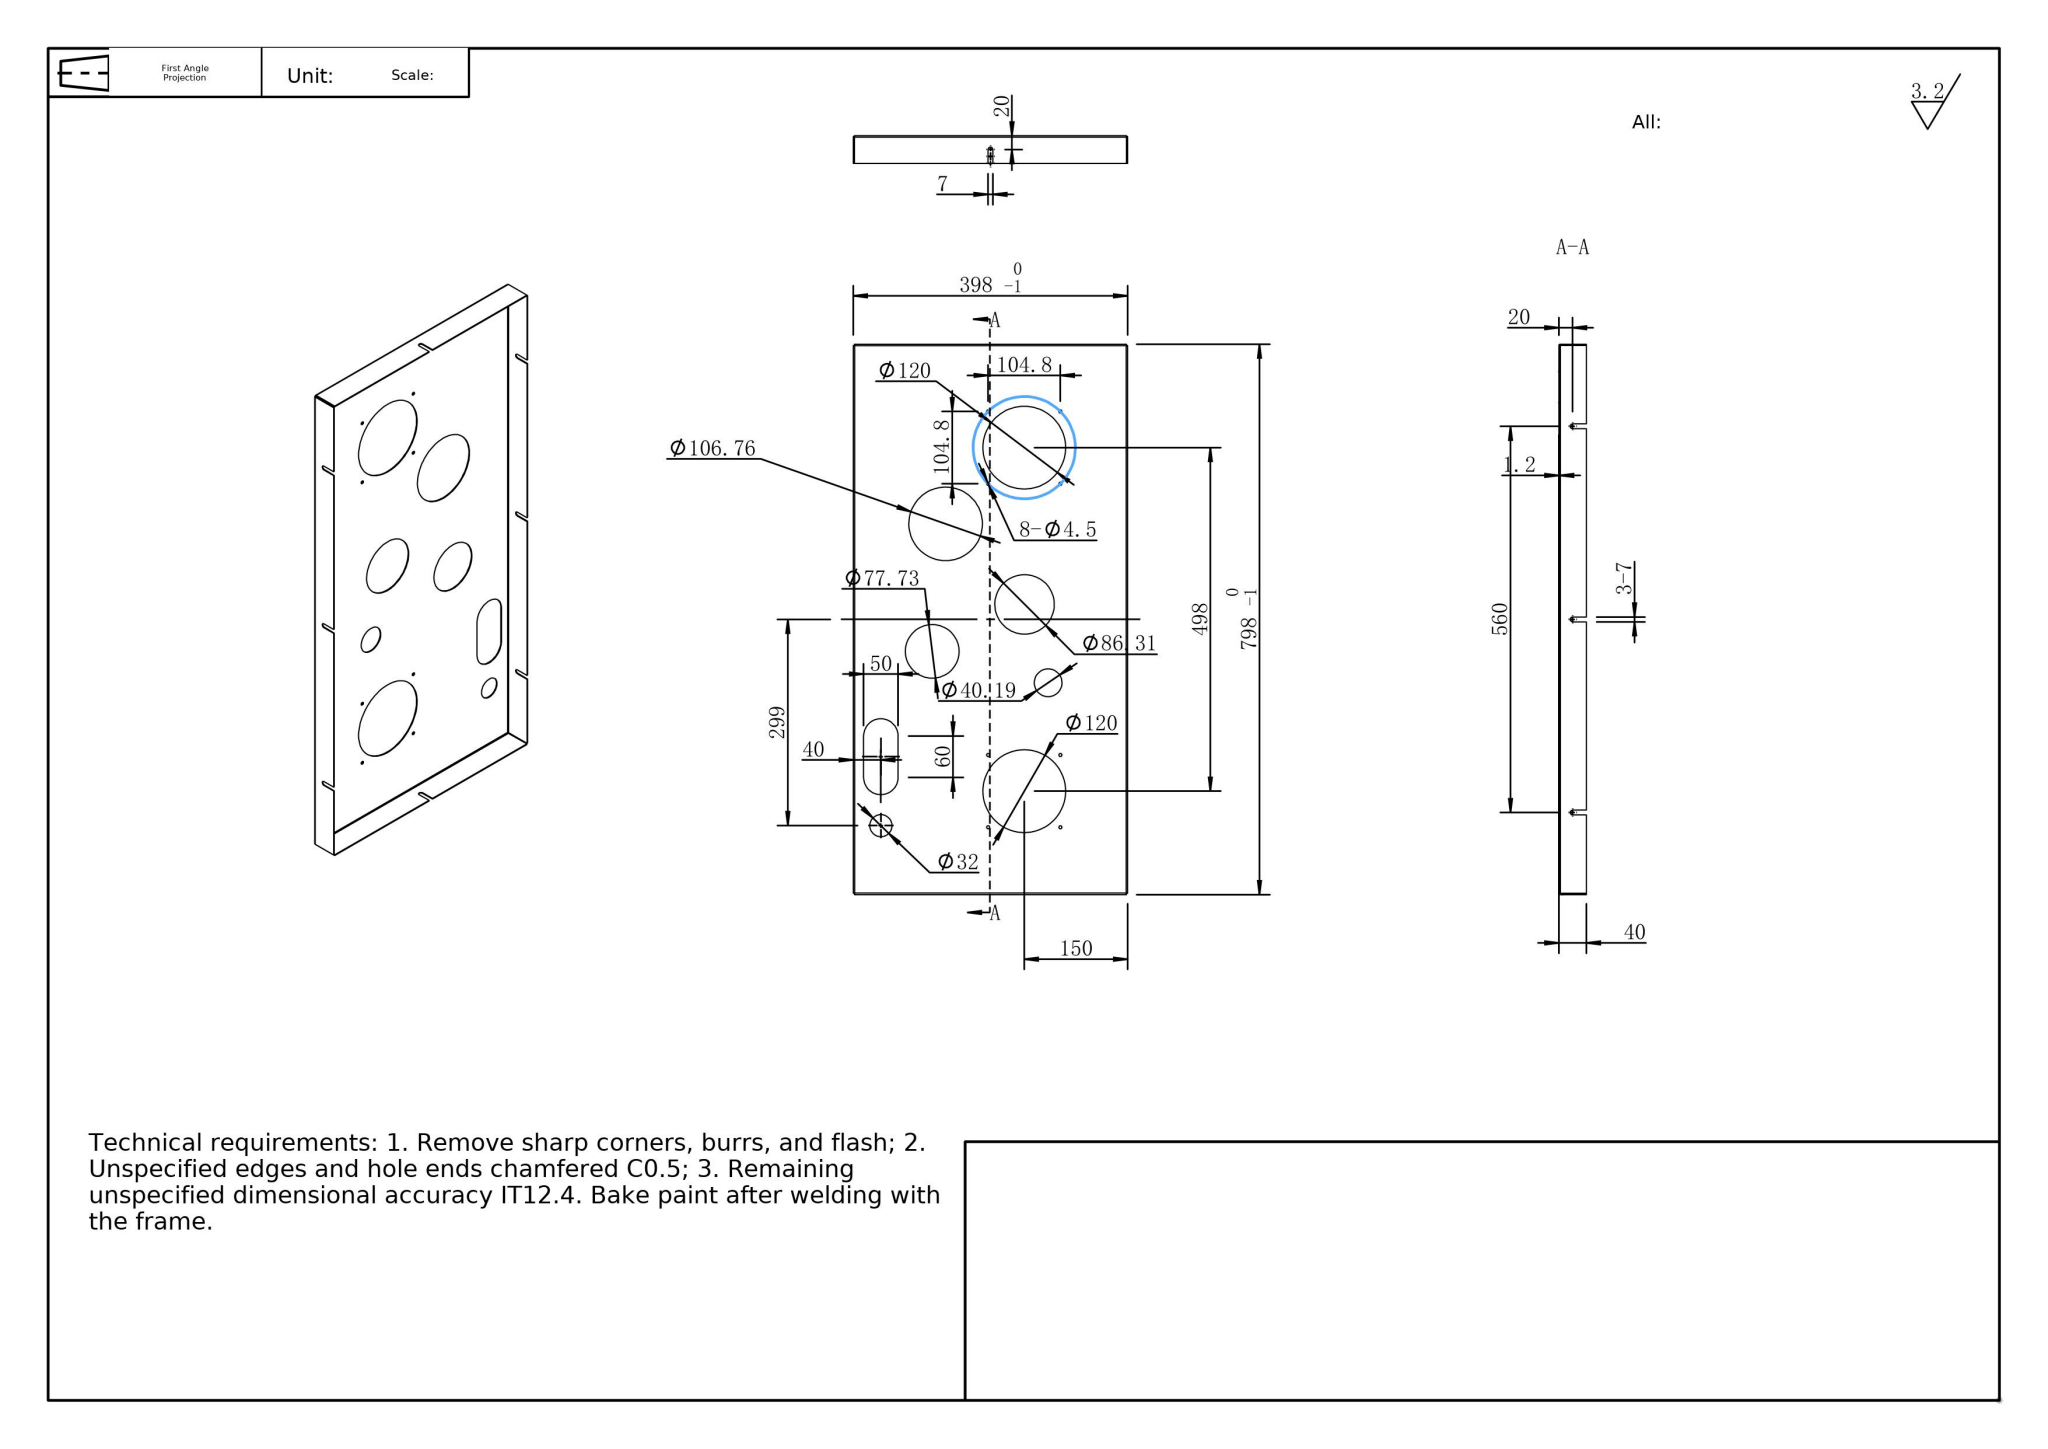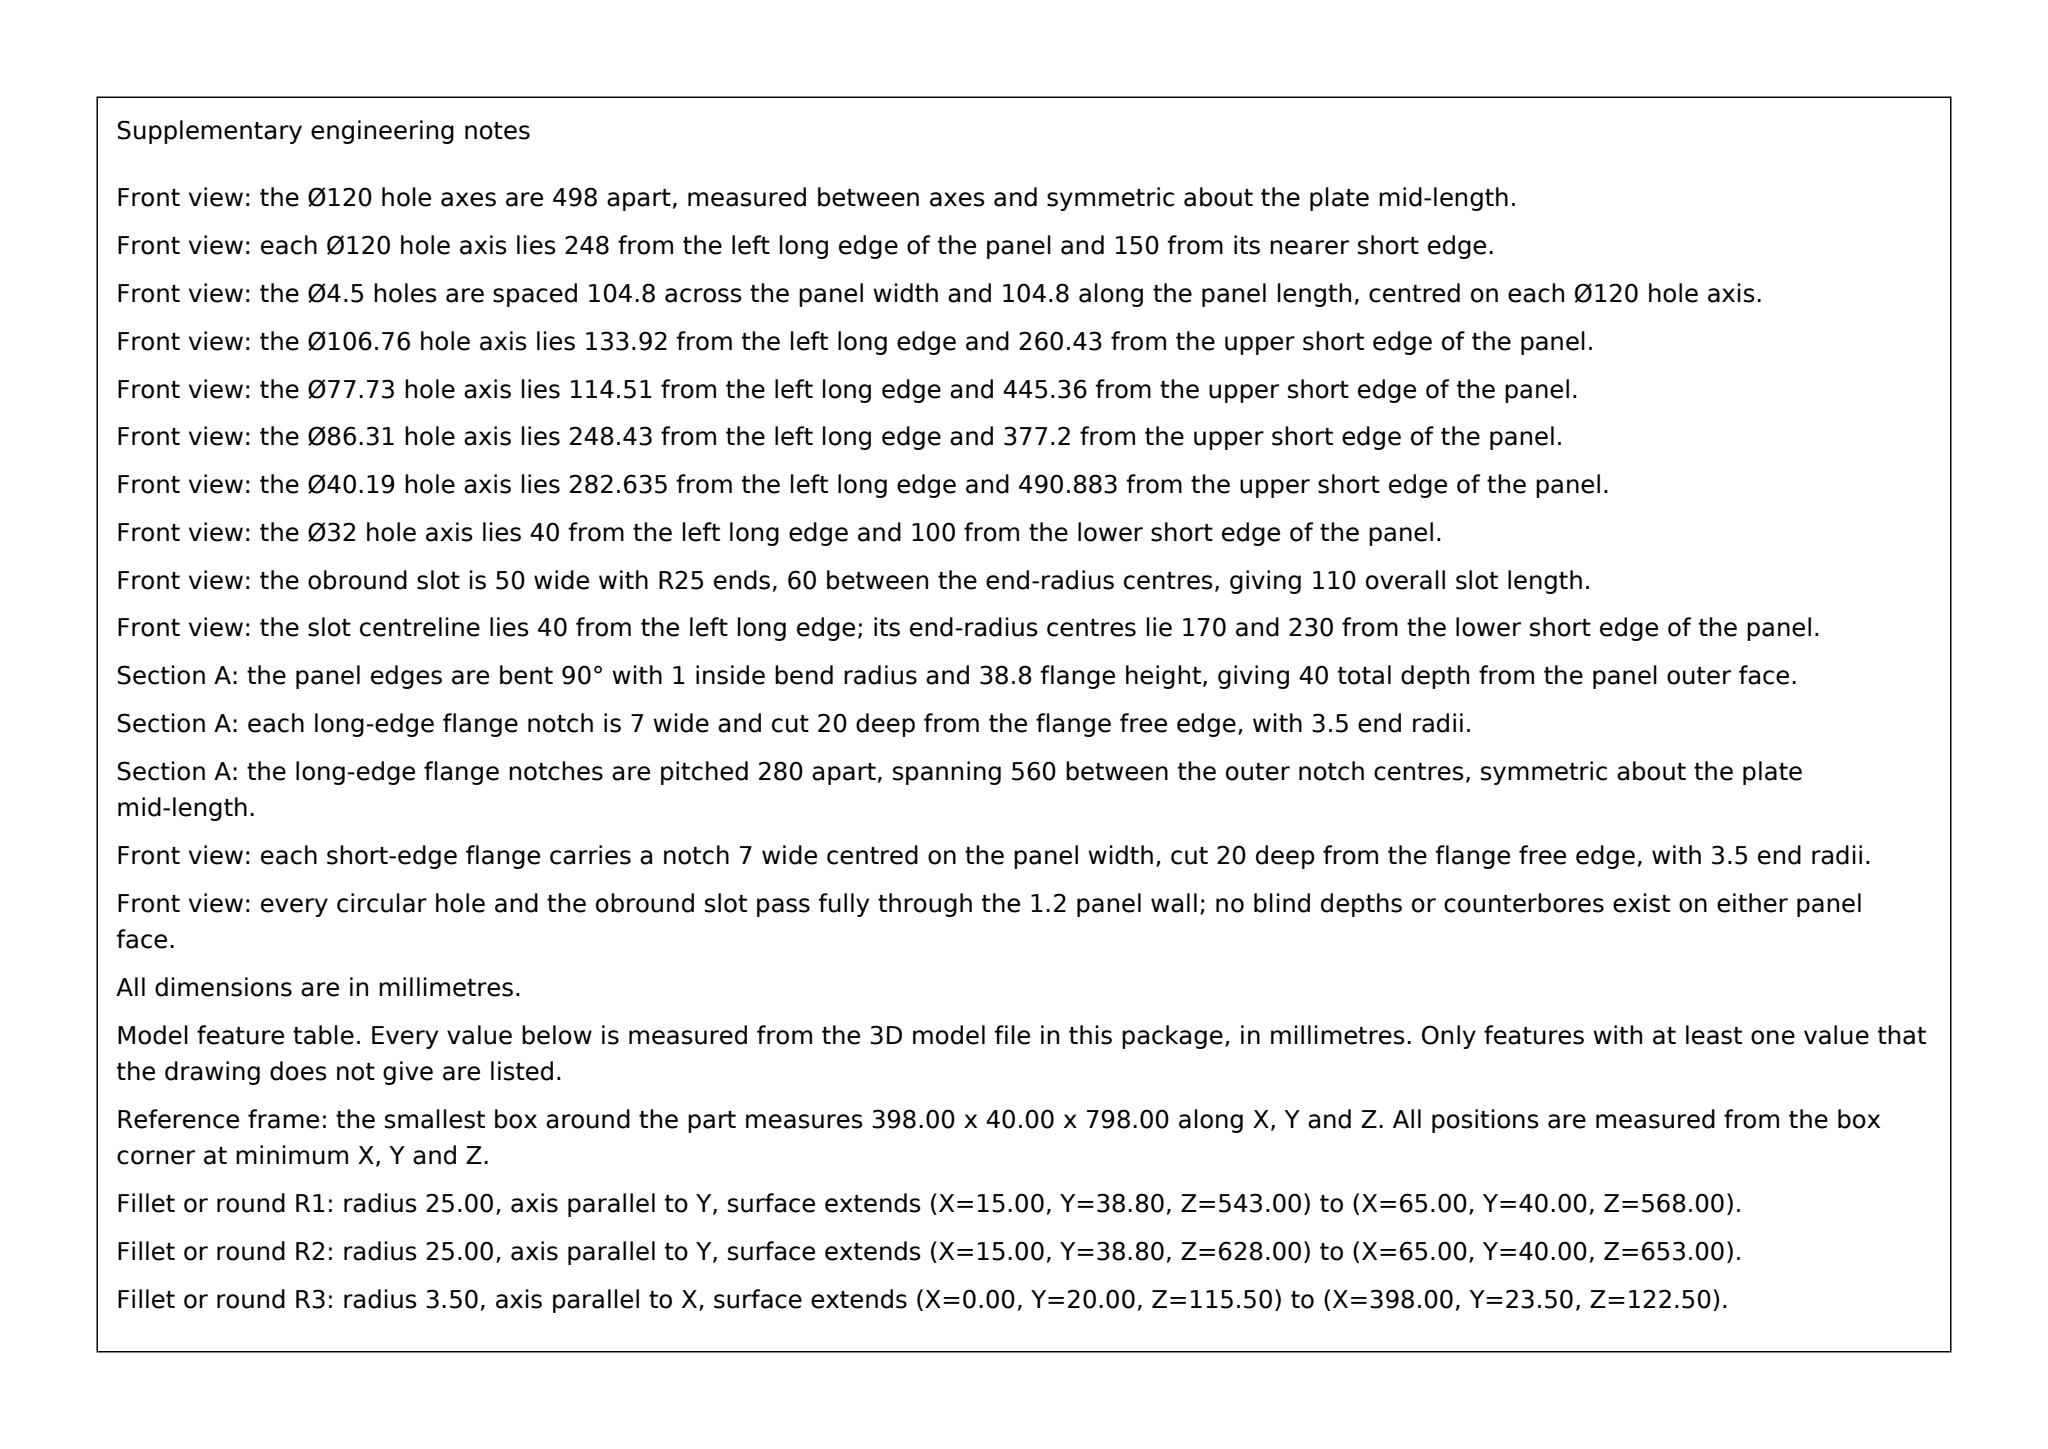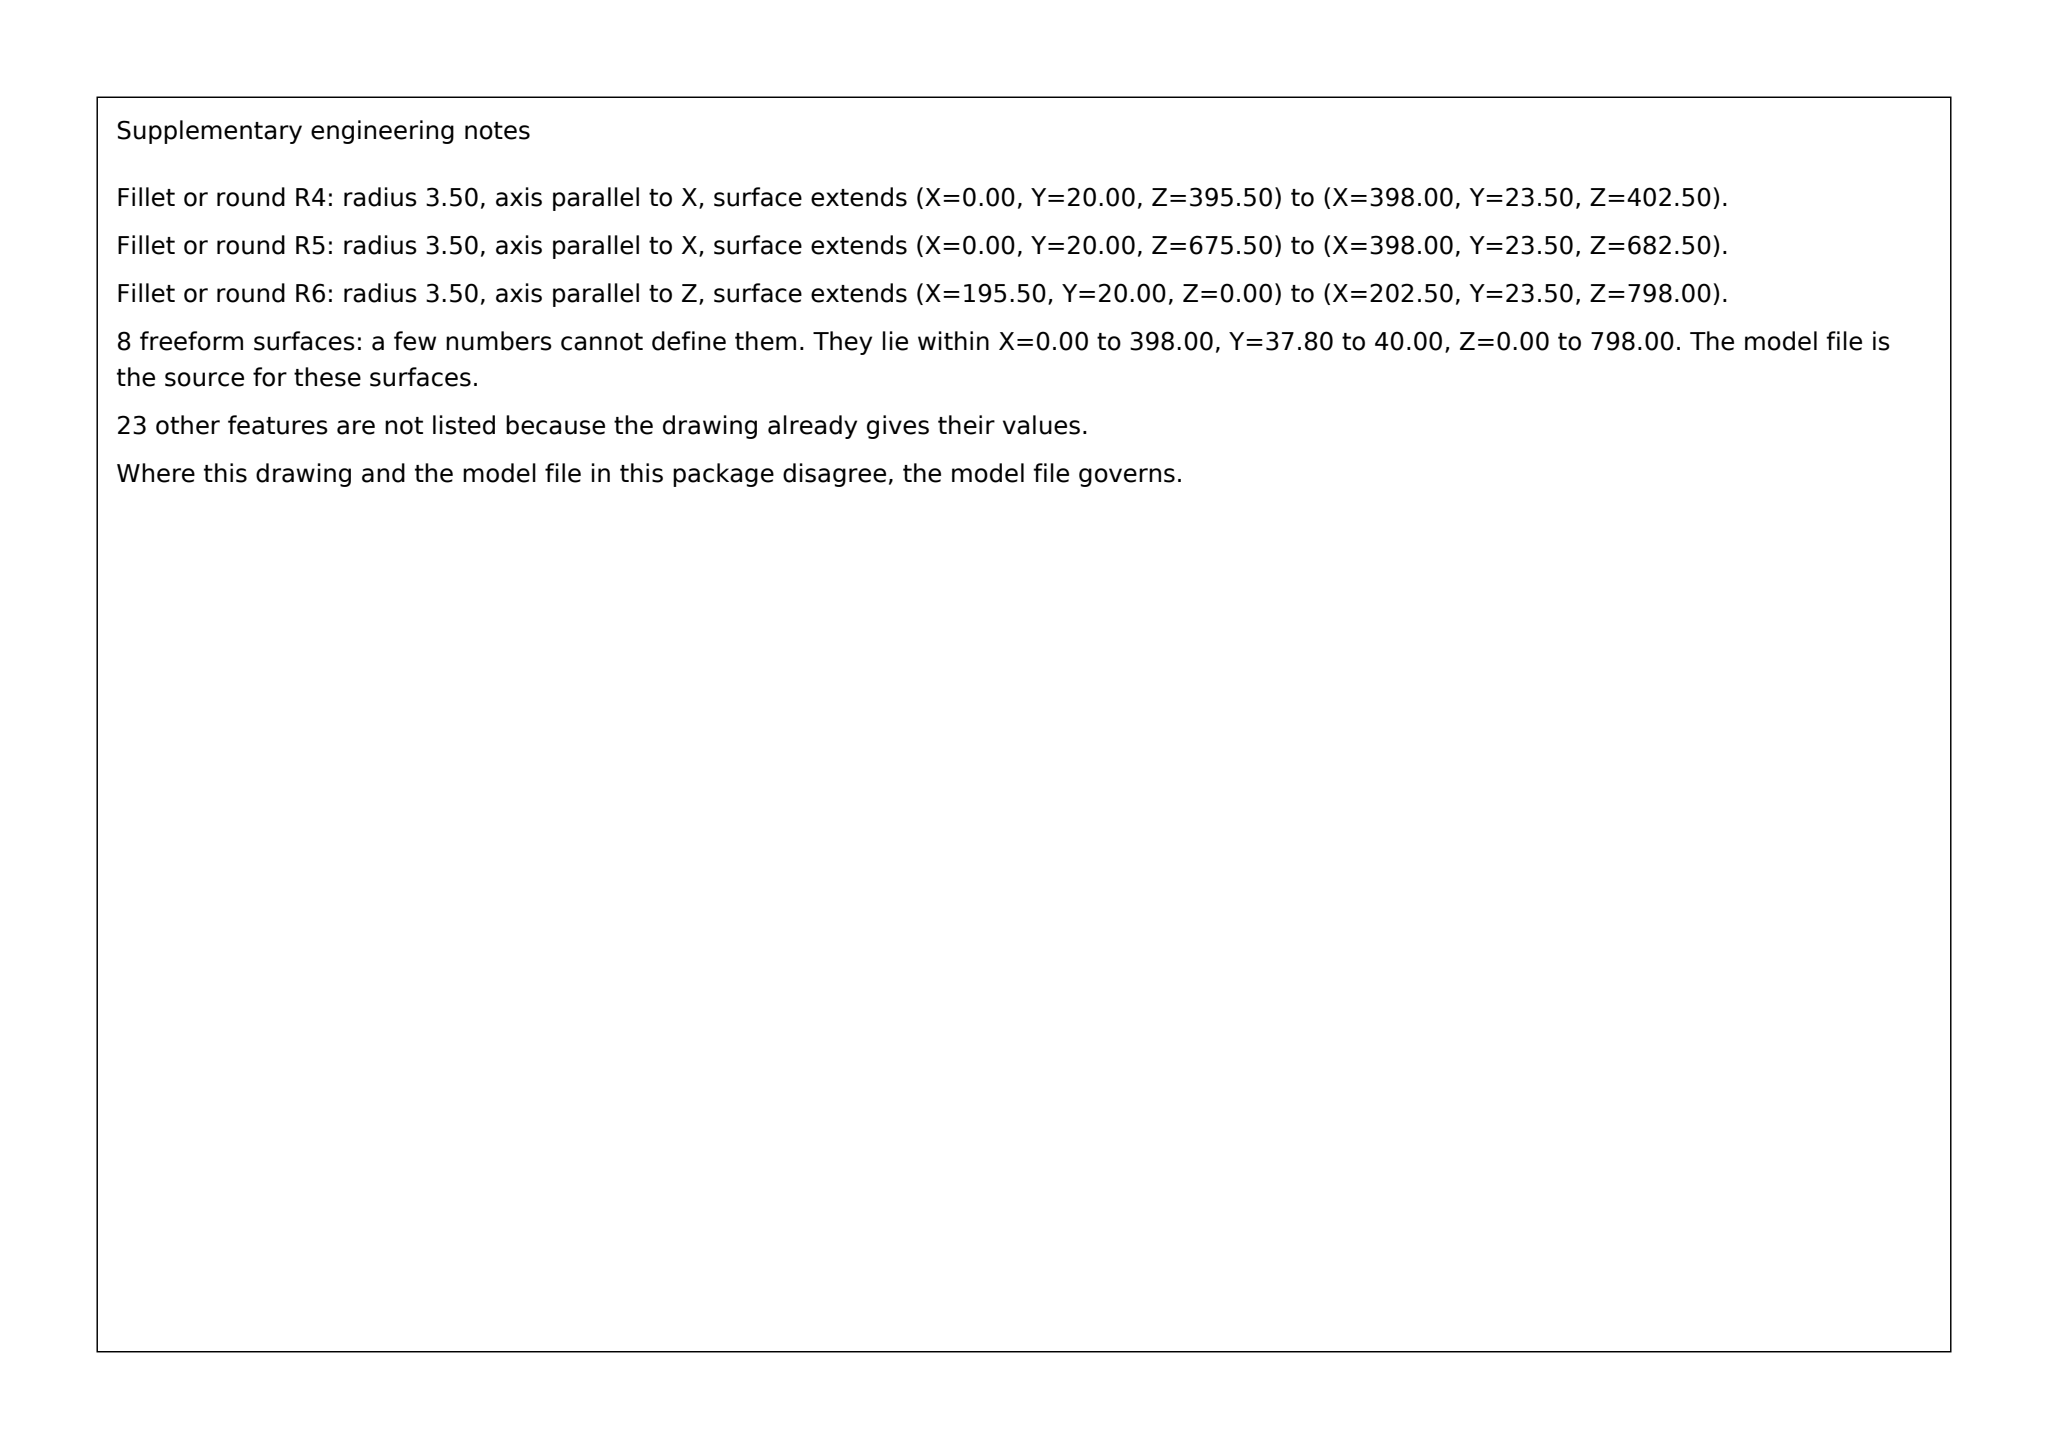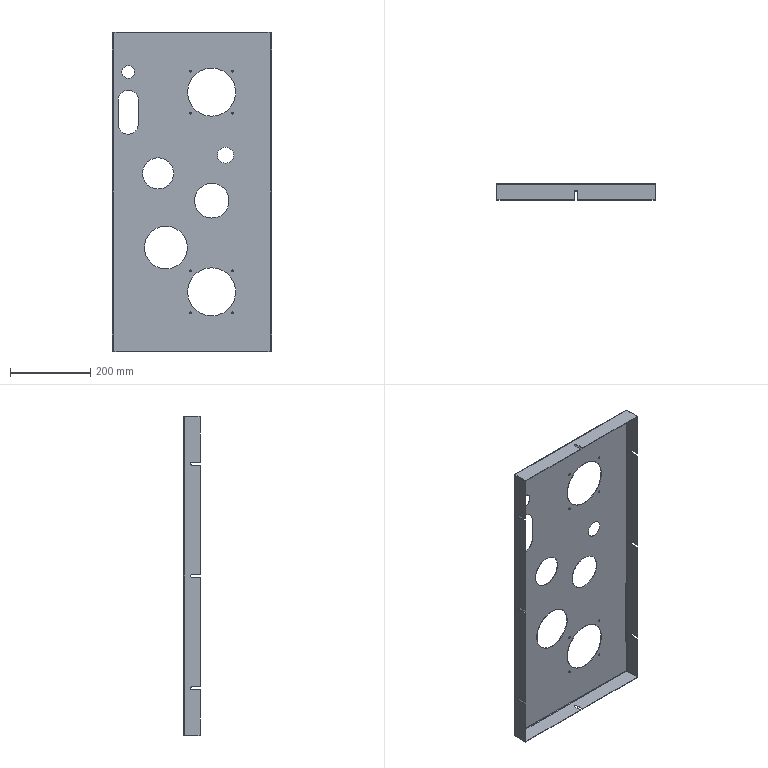Part | SolidWorks | mm | 1 solid | 113 faces | box 398 x 40 x 798 mm | volume 429082 mm3 | cylinder 57 | plane 48 | spline 8 | commonest cylinder face diameters 4.5 x16 7 x16 120 x4 4.4 x4 2 x4 50 x3 106.759 x2 77.727 x2
Drawing notes:
Ø106.76 CL: 133.94 FROM LEFT EDGE, 260.44 FROM BTM EDGE | from the solid: cyl dia 106.759 axis y at x=133.94, z=260.44 (bbox 398.024 x 798.024)
Ø77.73 CL: 114.52 FROM LEFT EDGE, 445.37 FROM BTM EDGE | from the solid: cyl dia 77.727 axis y at x=114.52, z=445.37
Ø86.31 CL: 248.44 FROM LEFT EDGE, 377.21 FROM BTM EDGE | from the solid: cyl dia 86.307 axis y at x=248.44, z=377.21
Ø40.19 CL: 282.65 FROM LEFT EDGE, 490.89 FROM BTM EDGE | from the solid: cyl dia 40.192 axis y at x=282.65, z=490.89
SLOT CL 40.01 FROM LEFT EDGE; END CTRS 568.01/628.01 FROM BTM | from the solid: two dia 50 cyls axis y at x=40.01, z=568.01 & 628.01 (60 apart)
Ø32 CL: 40.01 FROM LEFT EDGE, 698.01 FROM BTM EDGE | from the solid: cyl dia 32 axis y at x=40.01, z=698.01; same x as slot
FORMED FLANGES: R1 INSIDE, R2.2 OUTSIDE, TYP 4 PLCS | from the solid: bend cyls dia 2.0 (R1) and dia 4.4 (R2.2) along x and z at 4 edges
3-Ø7 IN SIDE FLANGE: 20 FROM FREE EDGE, 119.01 FROM END, 280 PITCH | from the solid: dia 7 axis x at y=20, z=119.01/399.01/679.01 (560 overall)
Ø7 IN END FLANGE: 199.01 FROM LEFT EDGE, 20 FROM FREE EDGE | from the solid: dia 7 axis z at x=199.01, y=20
Ø120 HOLES: CL 150 FROM EACH END EDGE, 498 APART | from the solid: Ø120 cyl axis Y at z=150.01 and z=648.01; bbox z=0.01..798.01; 648.01-150.01=498
3-Ø7 IN SIDE FLANGE 2 PLCS; Ø7 IN END FLANGE 2 PLCS; 8 TOTAL | from the solid: Ø7 axis-X holes at z=119.01/399.01/679.01 in both x=0 & x=398 flanges; Ø7 axis-Z holes at x=199.01 in both z=0 & z=798 flanges